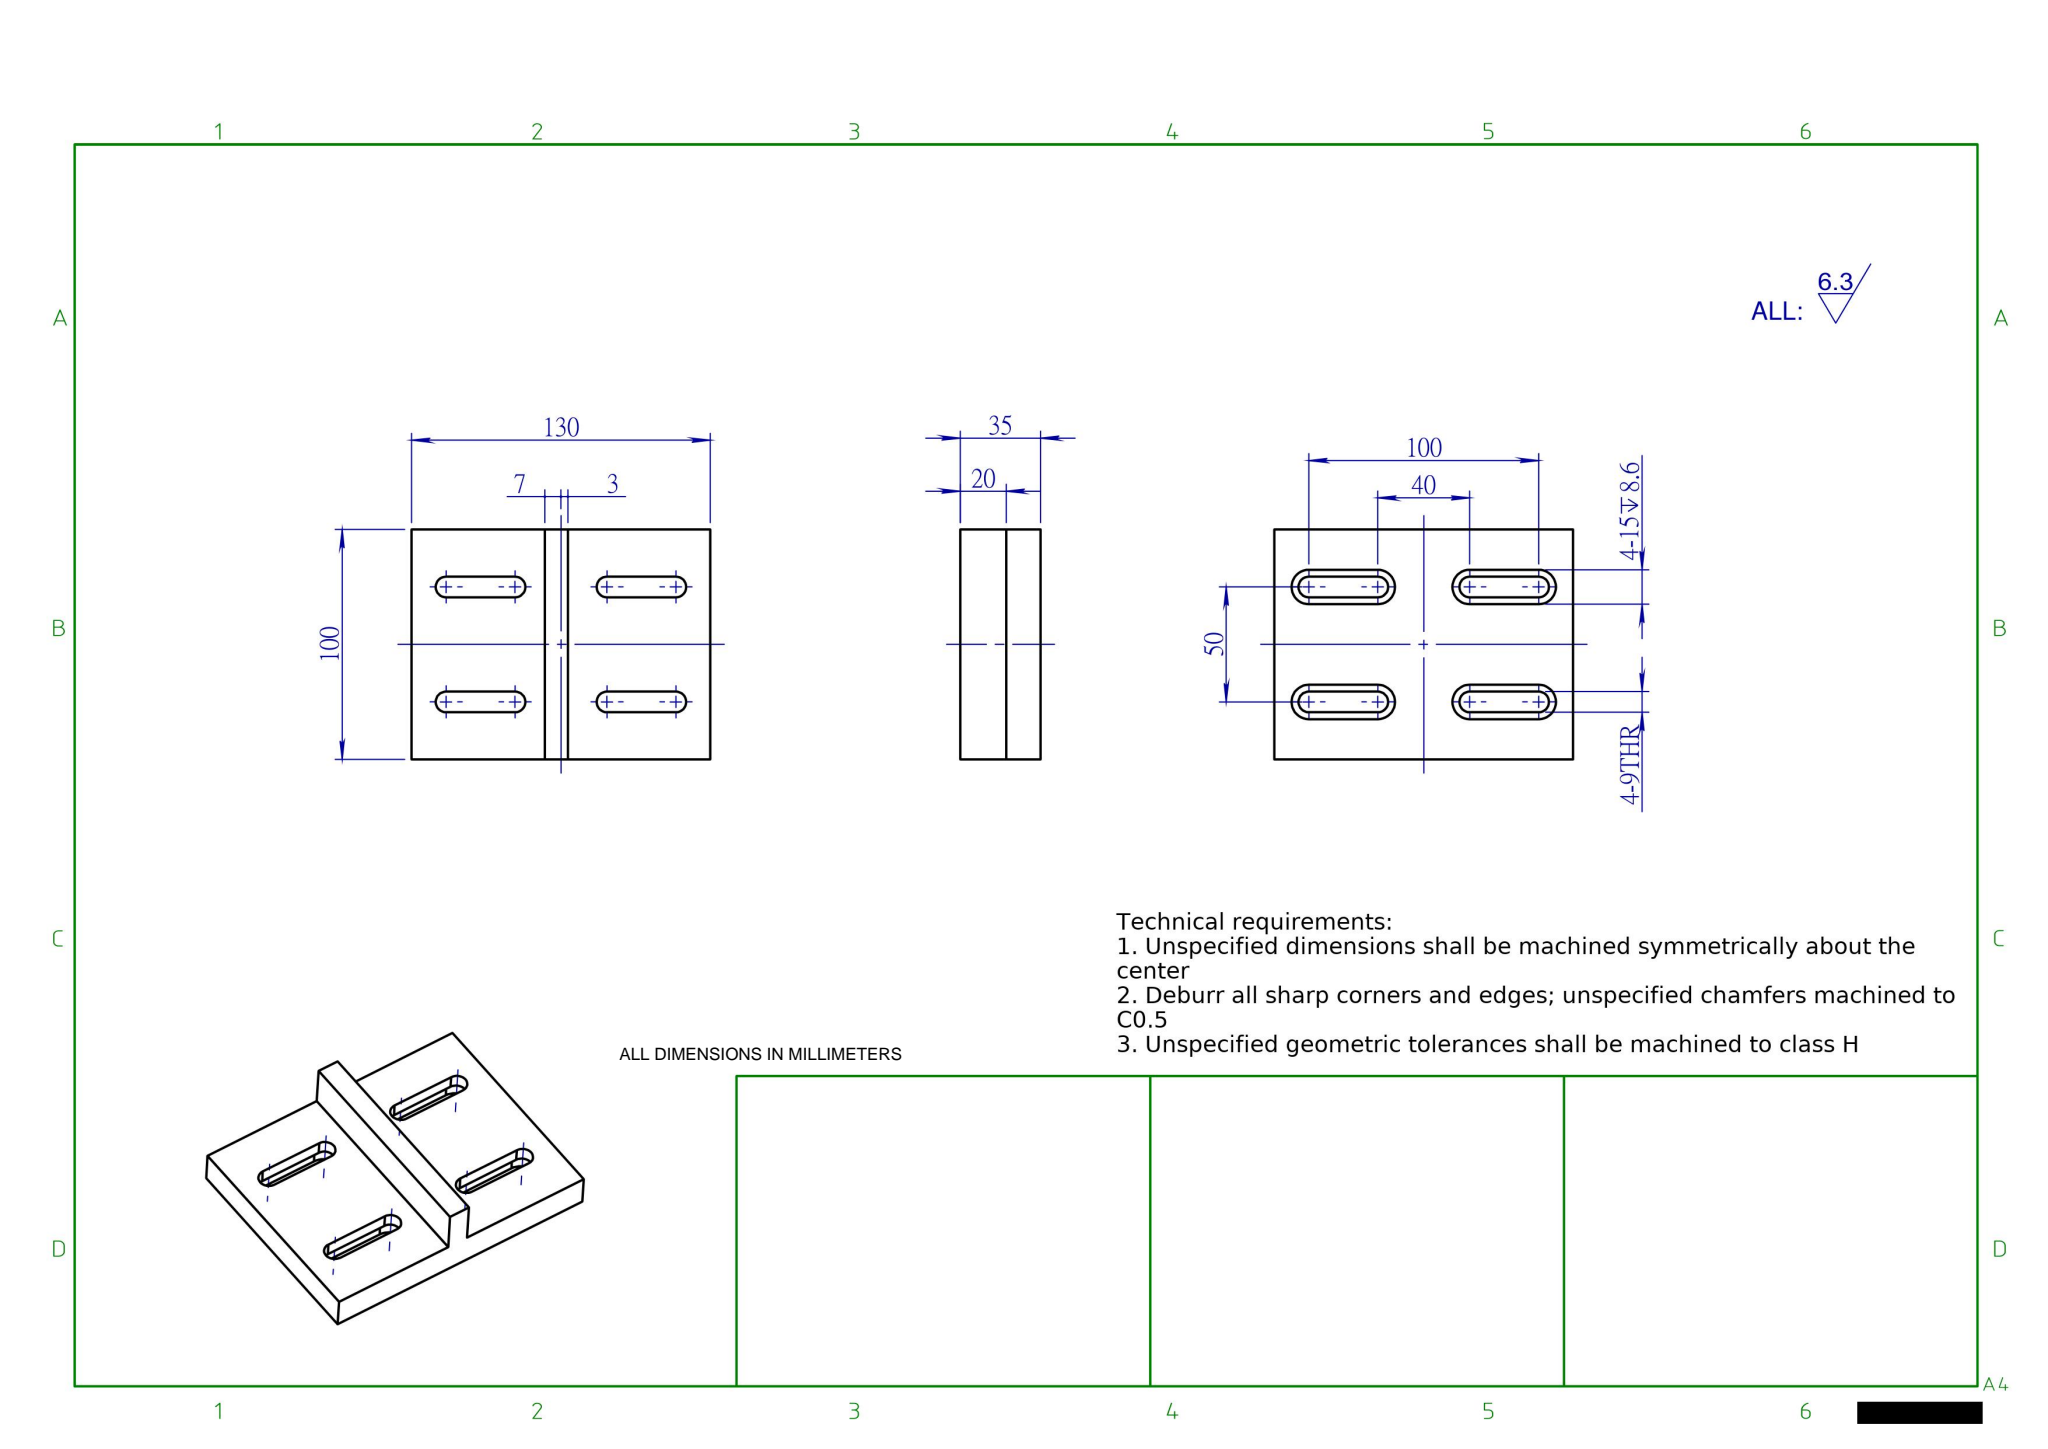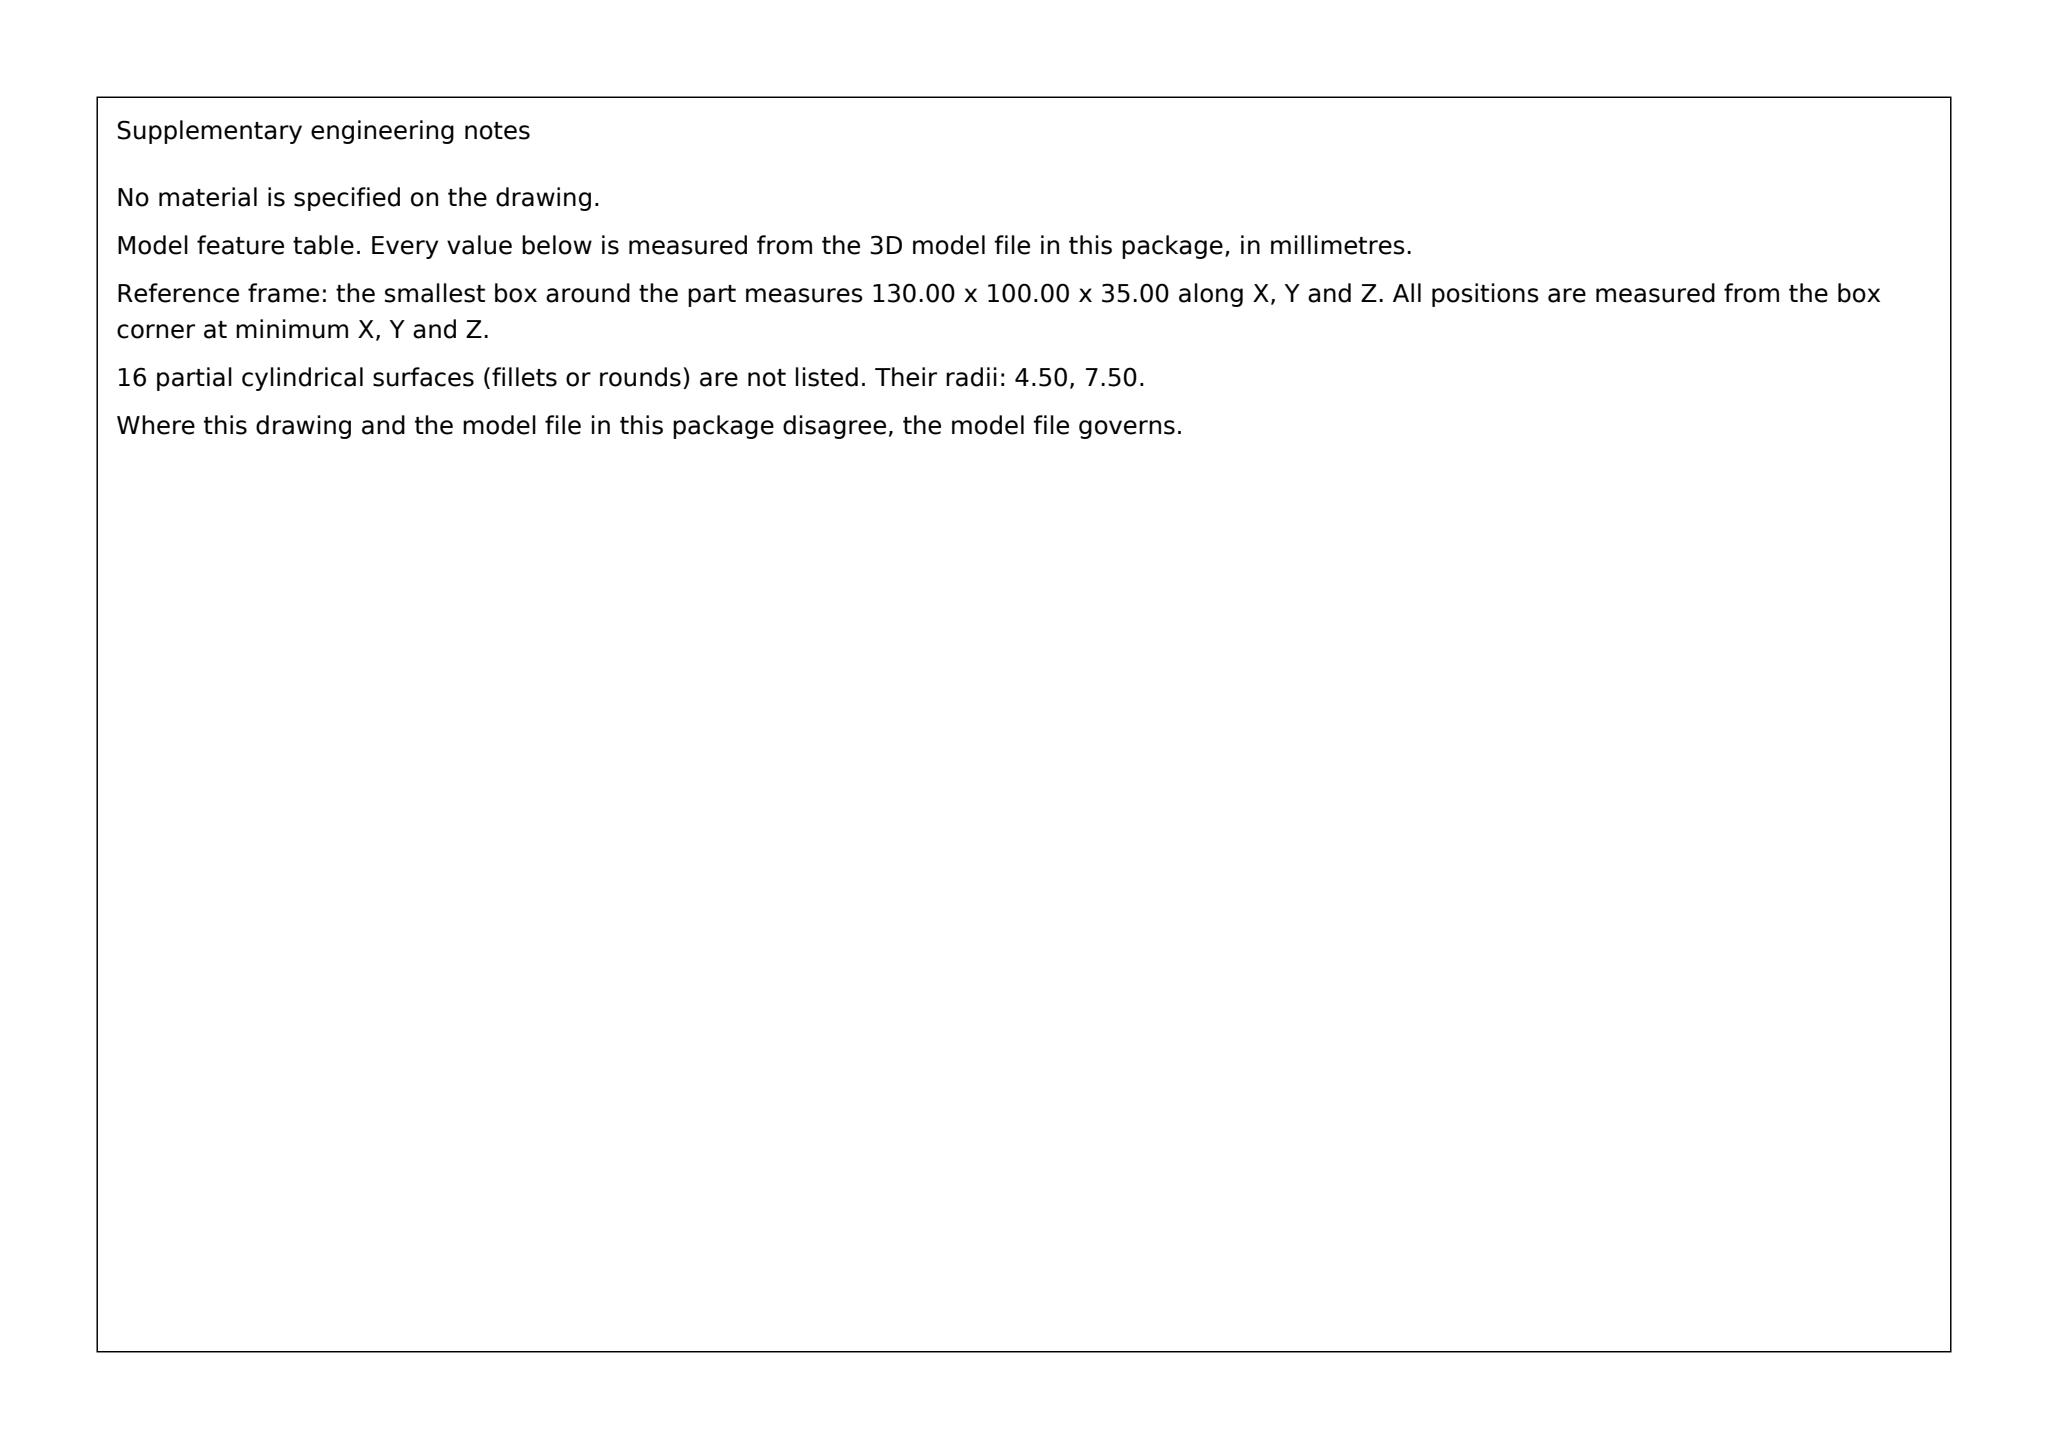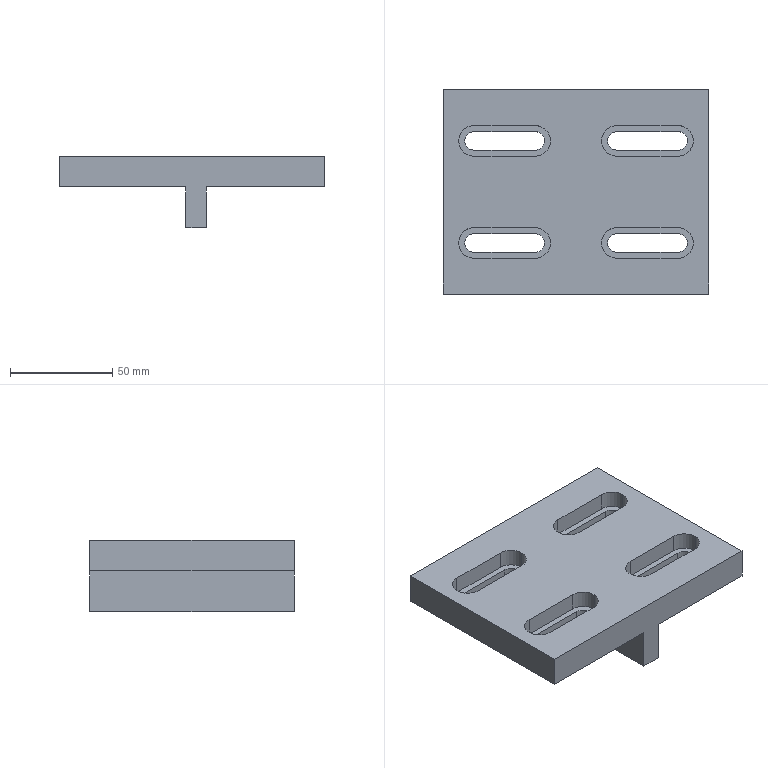Part | SolidWorks | mm | 1 solid | 54 faces | box 130 x 100 x 35 mm | volume 184900 mm3 | plane 30 | cylinder 24 | commonest cylinder face diameters 9 x12 15 x12
build123d program:
from build123d import *

# Parameters (mm, degrees)
SKETCH1_W                                            = 130
SKETCH1_H                                            = 100
BOSS_EXTRUDE1_DEPTH                                  = 7.5
COUNTERBORE_FOR_M8_HEX_SOCKET_HEAD_CAP_S_D           = 9
COUNTERBORE_FOR_M8_HEX_SOCKET_HEAD_CAP_S_CBORE_D     = 15
COUNTERBORE_FOR_M8_HEX_SOCKET_HEAD_CAP_S_CBORE_DEPTH = 8.6
CUT_EXTRUDE1_DEPTH                                   = 8.6
CUT_EXTRUDE2_DEPTH                                   = 83.456
SKETCH7_W                                            = 10
SKETCH7_H                                            = 100
BOSS_EXTRUDE2_DEPTH                                  = 20


with BuildPart() as part:
    # Sketch1 → Boss-Extrude1 (new, symmetric)
    with BuildSketch(Plane.XY):
        Rectangle(SKETCH1_W, SKETCH1_H)
    extrude(amount=BOSS_EXTRUDE1_DEPTH, both=True)

    # Counterbore for M8 Hex Socket Head Cap S (through all)
    with Locations(Plane.XY.offset(7.5)):
        with Locations((-50, 25), (-20, 25), (-50, -25), (-20, -25)):
            CounterBoreHole(COUNTERBORE_FOR_M8_HEX_SOCKET_HEAD_CAP_S_D / 2, COUNTERBORE_FOR_M8_HEX_SOCKET_HEAD_CAP_S_CBORE_D / 2, COUNTERBORE_FOR_M8_HEX_SOCKET_HEAD_CAP_S_CBORE_DEPTH)

    # Sketch4 → Cut-Extrude1 (cut)
    with BuildSketch(Plane.XY.offset(7.5)):
        with BuildLine():
            Line((-50, 32.5), (-20, 32.5))
            ThreePointArc((-20, 32.5), (-12.5, 25), (-20, 17.5))
            Line((-20, 17.5), (-50, 17.5))
            ThreePointArc((-50, 17.5), (-57.5, 25), (-50, 32.5))
        make_face()
        with BuildLine():
            Line((-50, -17.5), (-20, -17.5))
            ThreePointArc((-20, -17.5), (-12.5, -25), (-20, -32.5))
            Line((-20, -32.5), (-50, -32.5))
            ThreePointArc((-50, -32.5), (-57.5, -25), (-50, -17.5))
        make_face()
        with BuildLine():
            Line((20, 32.5), (50, 32.5))
            ThreePointArc((50, 32.5), (57.5, 25), (50, 17.5))
            Line((50, 17.5), (20, 17.5))
            ThreePointArc((20, 17.5), (12.5, 25), (20, 32.5))
        make_face()
        with BuildLine():
            Line((20, -17.5), (50, -17.5))
            ThreePointArc((50, -17.5), (57.5, -25), (50, -32.5))
            Line((50, -32.5), (20, -32.5))
            ThreePointArc((20, -32.5), (12.5, -25), (20, -17.5))
        make_face()
    extrude(amount=-CUT_EXTRUDE1_DEPTH, mode=Mode.SUBTRACT)

    # Sketch5 → Cut-Extrude2 (cut, through all)
    with BuildSketch(Plane.XY.offset(-1.1)):
        with BuildLine():
            Line((-50, 29.5), (-20, 29.5))
            ThreePointArc((-20, 29.5), (-15.5, 25), (-20, 20.5))
            Line((-20, 20.5), (-50, 20.5))
            ThreePointArc((-50, 20.5), (-54.5, 25), (-50, 29.5))
        make_face()
        with BuildLine():
            Line((-50, -20.5), (-20, -20.5))
            ThreePointArc((-20, -20.5), (-15.5, -25), (-20, -29.5))
            Line((-20, -29.5), (-50, -29.5))
            ThreePointArc((-50, -29.5), (-54.5, -25), (-50, -20.5))
        make_face()
        with BuildLine():
            Line((20, 29.5), (50, 29.5))
            ThreePointArc((50, 29.5), (54.5, 25), (50, 20.5))
            Line((50, 20.5), (20, 20.5))
            ThreePointArc((20, 20.5), (15.5, 25), (20, 29.5))
        make_face()
        with BuildLine():
            Line((20, -20.5), (50, -20.5))
            ThreePointArc((50, -20.5), (54.5, -25), (50, -29.5))
            Line((50, -29.5), (20, -29.5))
            ThreePointArc((20, -29.5), (15.5, -25), (20, -20.5))
        make_face()
    extrude(amount=-CUT_EXTRUDE2_DEPTH, mode=Mode.SUBTRACT)

    # Sketch7 → Boss-Extrude2 (add)
    with BuildSketch(Plane(origin=(0, 0, -7.5), x_dir=(-1, 0, 0), z_dir=(0, 0, -1))):
        with Locations((-2, 0)):
            Rectangle(SKETCH7_W, SKETCH7_H)
    extrude(amount=BOSS_EXTRUDE2_DEPTH)


solid = part.part